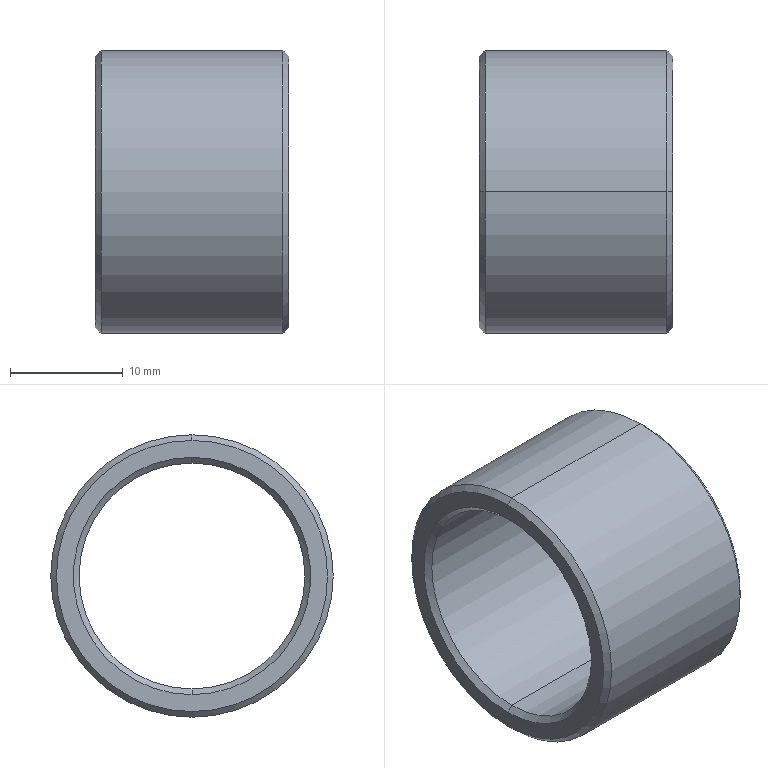Component | SolidWorks | ChainPartDriveShaftLocatingSleeve-1 | 1 solid | 14 faces | box 17.1 x 25 x 25 mm | volume 2986 mm3 | cone 8 | cylinder 4 | plane 2 | commonest cylinder face diameters 20 x2 25 x2
build123d program:
from build123d import *

# Parameters (mm, degrees)
SKETCH1_R           = 12.5
SKETCH1_R_2         = 10
BOSS_EXTRUDE1_DEPTH = 8.55
CHAMFER1_SIZE       = 0.5


with BuildPart() as part:
    # Sketch1 → Boss-Extrude1 (new, symmetric)
    with BuildSketch(Plane.XY):
        Circle(SKETCH1_R)
        Circle(SKETCH1_R_2, mode=Mode.SUBTRACT)
    extrude(amount=BOSS_EXTRUDE1_DEPTH, both=True)

    # Chamfer1
    chamfer1_edges = [part.edges().sort_by_distance(p)[0] for p in [
        (-12.5, 0, -8.55),
        (-12.5, 0, 8.55),
        (-10, 0, -8.55),
        (-10, 0, 8.55),
    ]]
    chamfer(chamfer1_edges, length=CHAMFER1_SIZE)


solid = part.part

# Placed as in the assembly
solid = solid.moved(Location((95.787, -2.563, -35.304), (0, 90, 0)))